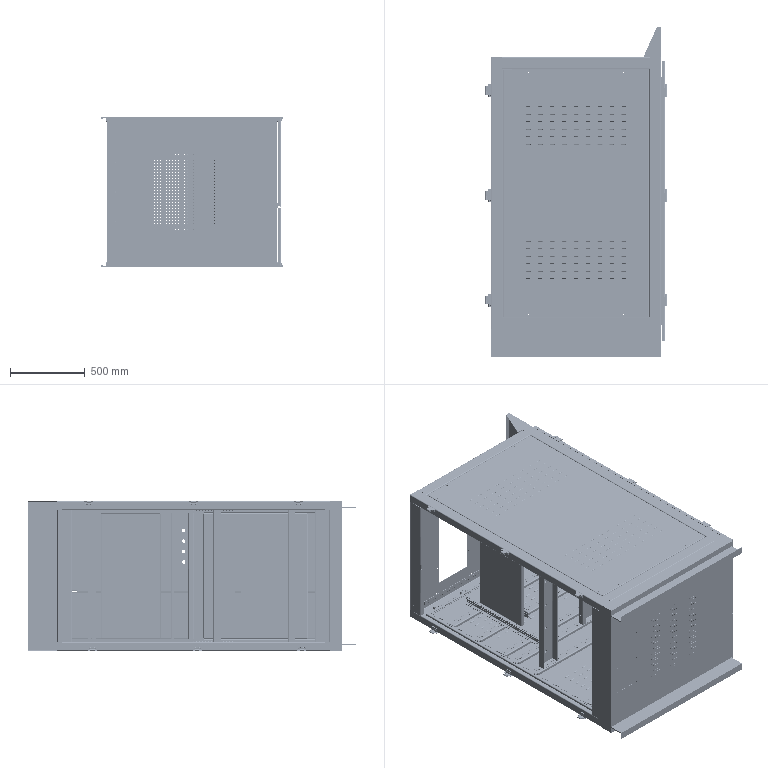Assembly | SolidWorks | mm | 113 component files | 113 solids | 13758 faces | box 1216 x 2200 x 1000 mm | volume 43776213 mm3 | cylinder 8078 | plane 4236 | sphere 864 | torus 432 | spline 100 | cone 48 | commonest cylinder face diameters 9 x4179 5 x1439 12 x336 6 x318 4 x286 16 x216 10 x210 14 x194
Bill of materials:
ACBMountingPlateF5 | 1 |  | Tall rectangular shallow tray/panel with bent perimeter flanges; flanges carry small holes along one long edge and on the short ends.
BaseCover | 1 |  | Rectangular flat panel with shallow return flanges around its edges and six round holes near the two long edges.
BottomSealingPlate | 1 |  | Thin flat rectangular sheet with a rectangular through-cutout, six small holes around the cutout, and a rectangular grid of small perforations.
10#ChannelSteel2 | 2 |  | Long straight U-shaped (channel) profile with no visible holes.
8#ChannelSteel1 | 2 |  | Long C-shaped channel with round holes in its web.
8#ChannelSteel2 | 2 |  | Long inverted-U channel whose top plate extends past the legs at both ends as flat tabs; one leg has a row of six round holes.
8#ChannelSteel3 | 2 |  | Long inverted-U channel similar to the previous part, with top-plate end tabs and two groups of four obround slots in one leg.
8#ChannelSteel5 | 1 |  | Plain long C-shaped channel with no visible holes.
BeamF1 | 12 |  | Long, shallow hat/U-shaped rail with rounded bends; the top web has a continuous row of round holes, and flat end tabs each carry two slots or holes.
BottomBeam | 1 |  | Tall bent sheet-metal profile: a C-section with rounded bends, unequal flanges and a return lip on one flange, with small holes and a small rectangular cutout.
BottomFrameCornerConnection | 2 |  | Flat L-shaped plate with rounded outer corners, a small inner-corner radius and three round through-holes.
Brow | 1 |  | Tall angled sheet-metal cover or wedge shape: two faces meet along a vertical edge, giving a right-trapezoid side profile; one face has small holes and slots.
CapacitorBeamF6 | 2 |  | Long, narrow rectangular tray or trough shape with an open face and closed end walls. It looks like a formed sheet channel.
CapacitorMountingPlateF6-00 | 1 |  | Flat rectangular sheet panel with formed C-shaped return flanges along two opposite edges.
Cover | 1 |  | Flat rectangular plate with one large rectangular cutout set off to one side and holes around the edge.
GL213-1Hinge1 | 6 |  | Block-shaped bracket with two raised, rounded lugs, each with a round through-bore, at either end of a lower connecting bar. It looks like a hinge-knuckle shape.
LeftFrontDoorPanel07-01 | 1 |  | Long, flat rectangular plate with two stacked rectangular windows, a column of round holes, a small slot near the bottom edge, and small hole pairs along the top edge.
MainMountingPlateF4-00 | 1 |  | Nearly square sheet panel with formed return flanges on two opposite edges and one long, narrow through-slot.
MiddleColumnF2-01 | 2 |  | Straight, perforated C-channel (U-channel) with rounded bends and evenly spaced round holes along the web and both flanges.
MiddleColumnF2 | 4 |  | Longer, perforated C-channel with the same profile as the shorter perforated channel. It has evenly spaced round holes along the web and flanges.
MirrorBottomBeam | 1 |  | Long formed sheet channel with an uneven C profile: one flange is short and one is long and ends in a return lip. A few holes run along one face.
MirrorBottomFrameCornerConnection | 2 |  | Flat L-shaped plate with rounded outer corners, a small inside corner radius, and three round through-holes.
MirrorTopBeamConnectionPlate | 2 |  | Flat L-shaped plate with rounded corners and three round through-holes. Its shape is similar to the other L-plate but in a different orientation, possibly mirrored.
MirrorUpperBeam | 1 |  | Long formed sheet post with a stepped profile: a box-like C-section plus an offset side flange. It has a row of small holes along one narrow face, a few larger holes, a small rectangular cutout or tab, and a hole near one end.
ProtectivePlate | 1 |  | Tall, narrow formed sheet-metal panel with several bends. A long flat web is bent into an angled upper section with a short vertical end lip. At the bottom is a horizontal foot leg with a small tab carrying one hole. One long edge flange has a row of small holes.
DoorRearVerticalStiffener06-1 | 2 |  | Long, slender formed rail with an open stepped profile that has rounded bends: a horizontal top flange, a vertical web, a horizontal step and a vertical lower leg. Many evenly spaced small holes run along its length, and there are small notches near the ends.
RightFrontDoorHorizontalStiffener06-02 | 2 |  | Short, straight formed channel section with an open multi-bend profile: two parallel long faces joined by a web, with an offset outer flange and rounded bends. One face has a column of larger round holes and the adjacent offset flange has two smaller holes.
RightFrontDoorPanel06-03 | 1 |  | Long, flat rectangular sheet panel with a narrow, slightly offset flange along one long edge. That flange is shorter than the panel at both ends. Small paired holes sit near the opposite long edge at three locations along the length.
BindingWireRack | 24 |  | U-shaped formed strap: a flat rectangular top web with one central round through-hole, and two parallel legs bent down at rounded corners.
GL213-1Hinge2 | 12 |  | Hinge-leaf-like bracket: a flat base plate with an upright plate that has two round holes and chamfered top corners. Along one edge is a cylindrical barrel (knuckle) with an axial through-bore, connected by a curved transition.
HBSW.001.001ColumnA | 2 |  | Long formed rail with an open profile: a deep C-section with rounded bends, plus a Z-offset step to an extra outward flange. One narrow flange has a dense row of small holes or slots along its length, and the web has a few small hole pairs and end holes.
HBSW.001.002ColumnB | 2 |  | Long formed rail similar in form to unnamed part but with the profile mirrored: an offset Z-step flange joined to a C-like section with rounded bends. One flange has a dense row of perforations, and there are small paired holes at three locations on the web.
HBSW.001.003SideTopBeam | 2 |  | Long formed rail with a multi-bend open profile (several 90-degree rounded bends, including a Z-step). The end tabs extend beyond the main body and carry round holes. One flange has a row of slotted/oblong perforations, and the web has a row of small holes with a few larger ones.
HBSW.001.004SideBottomBeam | 2 |  | Long formed rail with a C-section and a Z-offset extra flange, all with rounded bends. The outer web has six widely spaced elongated slots, the offset flange has a dense row of round holes, and the end tabs carry pairs of small holes.
LiftingRingReinforcementPlate | 4 |  | L-shaped angle bracket with a rounded inside bend. One leg has three equal round holes in a line. The other leg has a large central round hole flanked by two smaller round holes.
SidePlate | 2 |  | Thin, flat rectangular plate with two separate rectangular arrays of short slot-like features (about 9 columns by 6 rows each) near opposite ends, and small holes spaced around the perimeter.
SupportBeamF7 | 2 |  | Long, slender, straight bar or rail that looks like formed sheet. It has a single evenly spaced row of small round holes running along one narrow face. The end view shows a closed or channel-like profile with faceted, bent-looking corners and two large round holes on the end face.
TopBeamConnectionPlate | 2 |  | Flat L-shaped plate of uniform thin thickness with three round through-holes: one near the corner, one at the end of the short leg, and one near the end of the long leg. Outer corners are rounded and the inside corner has a fillet.
UpperBeam | 1 |  | Long, straight, formed sheet profile with a constant cross-section. The section is roughly C-shaped: a long back wall, a top web, a short return flange at the bottom, and on the other side a downward step that ends in an outward flange, with rounded bends. One narrow flange has a long row of small holes with a few larger holes spaced among them. There is a single hole near one end on another face and a small notch partway along one edge.
Mates:
1. coincident | BaseAssembly-1/ChannelSteelAssembly-1/8#ChannelSteel2-2 face at (-409.218, -82.9, -600) dir (0, 0, -1) | SidePanelAssembly-1/HBSW.001.001ColumnA-1 face at (-337.218, 1817.1, -600) dir (0, 0, -1)
2. coincident | BaseAssembly-1/ChannelSteelAssembly-1/8#ChannelSteel2-2 face at (-409.218, -2.9, -600) dir (0, 1, 0) | SidePanelAssembly-1/HBSW.001.004SideBottomBeam-1 face at (-413.718, -2.9, -600) dir (0, -1, 0)
3. coincident | BaseAssembly-1/ChannelSteelAssembly-1/8#ChannelSteel1-2 face at (722.782, -82.9, -600) dir (1, 0, 0) | SidePanelAssembly-1/HBSW.001.002ColumnB-1 face at (722.782, 1817.1, -597) dir (1, 0, 0)
4. coincident | BaseAssembly-1/ChannelSteelAssembly-1/8#ChannelSteel1-1 face at (-417.218, -82.9, 400) dir (-1, 0, 0) | SidePanelAssembly-2/HBSW.001.002ColumnB-1 face at (-417.218, 1817.1, 397) dir (-1, 0, 0)
5. coincident | BaseAssembly-1/ChannelSteelAssembly-1/8#ChannelSteel2-1 face at (714.782, -2.9, 400) dir (0, 1, 0) | SidePanelAssembly-2/HBSW.001.004SideBottomBeam-1 face at (719.282, -2.9, 400) dir (0, -1, 0)
6. coincident | BaseAssembly-1/ChannelSteelAssembly-1/8#ChannelSteel2-1 face at (714.782, -82.9, 400) dir (0, 0, 1) | SidePanelAssembly-2/HBSW.001.004SideBottomBeam-1 face at (-339.718, 77.1, 400) dir (0, 0, 1)
7. concentric | SidePanelAssembly-2/HBSW.001.004SideBottomBeam-1 face at (-372.218, 17.1, 352) dir (0, 0, -1) r 5.5 | BottomBeamAssembly-1/BottomFrameCornerConnection-2 face at (-372.218, 17.1, 332) dir (0, 0, 1) r 5.75
8. concentric | SidePanelAssembly-2/HBSW.001.004SideBottomBeam-1 face at (-397.218, 17.1, 352) dir (0, 0, -1) r 5.5 | BottomBeamAssembly-1/BottomFrameCornerConnection-2 face at (-397.218, 17.1, 332) dir (0, 0, 1) r 5.75
9. coincident | SidePanelAssembly-2/HBSW.001.002ColumnB-1 edge at (-411.218, 27.6, 342) dir (0, 1, 0) | BottomBeamAssembly-1/BottomFrameCornerConnection-2 face at (-414.218, 0.09974, 342) dir (0, 0, 1)
10. concentric | SidePanelAssembly-1/HBSW.001.004SideBottomBeam-1 face at (677.782, 17.1, -552) dir (0, 0, 1) r 5.5 | MirrorBottomBeamAssembly-2/MirrorBottomFrameCornerConnection-1 face at (677.782, 17.1, -549) dir (0, 0, 1) r 5.75
11. concentric | SidePanelAssembly-1/HBSW.001.004SideBottomBeam-1 face at (702.782, 17.1, -552) dir (0, 0, 1) r 5.5 | MirrorBottomBeamAssembly-2/MirrorBottomFrameCornerConnection-1 face at (702.782, 17.1, -549) dir (0, 0, 1) r 5.75
12. coincident | SidePanelAssembly-1/HBSW.001.002ColumnB-1 face at (719.782, 1786.6, -542) dir (0, 0, 1) | MirrorBottomBeamAssembly-2/MirrorBottomFrameCornerConnection-1 face at (719.782, 0.09974, -542) dir (0, 0, -1)
13. concentric | SidePanelAssembly-2/HBSW.001.003SideTopBeam-1 face at (-357.218, 1797.1, 352) dir (0, 0, -1) r 5.5 | TopBeamAssembly-1/TopBeamConnectionPlate-2 face at (-357.218, 1797.1, 349) dir (0, 0, -1) r 5.75
14. concentric | SidePanelAssembly-2/HBSW.001.003SideTopBeam-1 face at (-397.218, 1797.1, 352) dir (0, 0, -1) r 5.5 | TopBeamAssembly-1/TopBeamConnectionPlate-2 face at (-397.218, 1797.1, 349) dir (0, 0, -1) r 5.75
15. coincident | SidePanelAssembly-2/HBSW.001.003SideTopBeam-1 face at (-413.718, 1787.1, 342) dir (0, 0, -1) | TopBeamAssembly-1/TopBeamConnectionPlate-2 face at (-414.218, 1814.1, 342) dir (0, 0, 1)
16. concentric | SidePanelAssembly-1/HBSW.001.003SideTopBeam-1 face at (702.782, 1797.1, -552) dir (0, 0, 1) r 5.5 | MirrorTopBeamAssembly-2/MirrorTopBeamConnectionPlate-1 face at (702.782, 1797.1, -532) dir (0, 0, -1) r 5.75
17. concentric | SidePanelAssembly-1/HBSW.001.003SideTopBeam-1 face at (662.782, 1797.1, -552) dir (0, 0, 1) r 5.5 | MirrorTopBeamAssembly-2/MirrorTopBeamConnectionPlate-1 face at (662.782, 1797.1, -532) dir (0, 0, -1) r 5.75
18. coincident | SidePanelAssembly-1/HBSW.001.003SideTopBeam-1 face at (719.282, 1787.1, -542) dir (0, 0, 1) | MirrorTopBeamAssembly-2/MirrorTopBeamConnectionPlate-1 face at (719.782, 1814.1, -542) dir (0, 0, -1)
19. distance | SidePlate-1 face at (640.782, 1735.6, -597) dir (1, 0, 0) | SidePanelAssembly-1/HBSW.001.002ColumnB-1 face at (642.782, 77.6, -597) dir (-1, 0, 0)
20. distance | SidePanelAssembly-1/HBSW.001.004SideBottomBeam-1 face at (-339.718, 77.1, -597) dir (0, 1, 0) | SidePlate-1 face at (636.782, 78.6, -597) dir (0, -1, 0)
21. coincident | SidePanelAssembly-1/HBSW.001.001ColumnA-1 face at (-337.218, 77.6, -578) dir (0, 0, -1) | SidePlate-1 face at (-335.218, 1735.6, -578) dir (0, 0, 1)
22. distance | SidePlate-2 face at (-335.218, 78.6, 378) dir (-1, 0, 0) | SidePanelAssembly-2/HBSW.001.002ColumnB-1 face at (-337.218, 77.6, 397) dir (1, 0, 0)
23. distance | SidePlate-2 face at (636.782, 1735.6, 397) dir (0, 1, 0) | SidePanelAssembly-2/HBSW.001.003SideTopBeam-1 face at (-339.718, 1737.1, 397) dir (0, -1, 0)
24. coincident | SidePanelAssembly-2/HBSW.001.001ColumnA-1 face at (642.782, 77.6, 378) dir (0, 0, 1) | SidePlate-2 face at (640.782, 78.6, 378) dir (0, 0, -1)
25. distance | Cover-1 face at (640.782, 1790.1, 340) dir (0, 0, 1) | SidePanelAssembly-2/HBSW.001.003SideTopBeam-1 face at (-413.718, 1787.1, 342) dir (0, 0, -1)
26. distance | Cover-1 face at (-335.218, 1790.1, 336) dir (-1, 0, 0) | TopBeamAssembly-1/UpperBeam-1 face at (-337.218, 1817.1, 342) dir (1, 0, 0)
27. coincident | MirrorTopBeamAssembly-2/MirrorUpperBeam-1 face at (642.782, 1790.1, -542) dir (0, 1, 0) | Cover-1 face at (-335.218, 1790.1, -540) dir (0, -1, 0)
28. concentric | SidePanelAssembly-2/GL213-1Hinge2-1 face at (754.782, 1597.1, 394) dir (0, -1, 0) r 3 | LeftFrontDoorAssembly-1/GL213-1Hinge1-1 face at (754.782, 1612.1, 394) dir (0, -1, 0) r 3
29. coincident | SidePanelAssembly-2/GL213-1Hinge2-1 face at (754.782, 1597.1, 400) dir (0, 1, 0) | LeftFrontDoorAssembly-1/GL213-1Hinge1-1 face at (814.782, 1597.1, 400) dir (0, -1, 0)
30. concentric | SidePanelAssembly-1/GL213-1Hinge2-5 face at (754.782, 1592.1, -594) dir (0, 1, 0) r 3 | RightFrontDoorAssembly-1/GL213-1Hinge1-3 face at (754.782, 1577.1, -594) dir (0, 1, 0) r 3
31. coincident | SidePanelAssembly-1/GL213-1Hinge2-5 face at (754.782, 1622.1, -600) dir (0, 1, 0) | RightFrontDoorAssembly-1/GL213-1Hinge1-3 face at (814.782, 1622.1, -600) dir (0, -1, 0)
32. coincident | LeftFrontDoorAssembly-1/LeftFrontDoorPanel07-01-1 face at (747.782, 857.1, 98.5) dir (1, 0, 0) | RightFrontDoorAssembly-1/RightFrontDoorPanel06-03-1 face at (747.782, 857.1, -401) dir (1, 0, 0)
33. concentric | SidePanelAssembly-1/HBSW.001.002ColumnB-1 face at (625.282, 257.1, -585) dir (0, 0, 1) r 4.5 | BeamF1-2 face at (625.282, 257.1, -582) dir (0, 0, 1) r 4.5
34. coincident | SidePanelAssembly-1/HBSW.001.002ColumnB-1 face at (642.782, 1736.6, -575) dir (0, 0, 1) | BeamF1-2 face at (152.782, 247.1, -575) dir (0, 0, -1)
35. concentric | SidePanelAssembly-1/HBSW.001.001ColumnA-1 face at (-319.718, 257.1, -585) dir (0, 0, 1) r 4.5 | BeamF1-2 face at (-319.718, 257.1, -582) dir (0, 0, 1) r 4.5
36. coincident | SidePanelAssembly-2/HBSW.001.001ColumnA-1 face at (642.782, 77.6, 375) dir (0, 0, -1) | BeamF1-14 face at (152.782, 247.1, 375) dir (0, 0, 1)
37. concentric | SidePanelAssembly-2/HBSW.001.001ColumnA-1 face at (625.282, 257.1, 385) dir (0, 0, -1) r 4.5 | BeamF1-14 face at (625.282, 257.1, 382) dir (0, 0, -1) r 4.5
38. concentric | SidePanelAssembly-2/HBSW.001.002ColumnB-1 face at (-319.718, 257.1, 385) dir (0, 0, -1) r 4.5 | BeamF1-14 face at (-319.718, 257.1, 382) dir (0, 0, -1) r 4.5
39. coincident | BeamF1-15 face at (152.782, 747.1, 372) dir (0, 0, -1) | MiddleColumnF2-1 face at (517.782, 497.1, 372) dir (0, 0, 1)
40. concentric | BeamF1-15 face at (532.782, 747.1, 382) dir (0, 0, -1) r 4.5 | MiddleColumnF2-1 face at (532.782, 747.1, 372) dir (0, 0, -1) r 4.5
41. concentric | BeamF1-14 face at (532.782, 247.1, 382) dir (0, 0, -1) r 4.5 | MiddleColumnF2-1 face at (532.782, 247.1, 372) dir (0, 0, -1) r 4.5
42. distance | ACBMountingPlateF5-1 face at (452.782, 942.1, -571) dir (0, 0, -1) | BeamF1-7 face at (152.782, 927.1, -572) dir (0, 0, 1)
43. concentric | BeamF1-16 face at (572.782, 927.1, 382) dir (0, 0, -1) r 4.5 | ACBMountingPlateF5-1 face at (572.782, 927.1, 371.008) dir (0, 0, -1) r 4.5
44. concentric | BeamF1-16 face at (452.782, 927.1, 382) dir (0, 0, -1) r 4.5 | ACBMountingPlateF5-1 face at (452.782, 927.1, 371.008) dir (0, 0, -1) r 4.5
45. distance | CapacitorBeamF6-1 face at (-177.218, 275.1, -571) dir (0, 0, -1) | BeamF1-2 face at (152.782, 247.1, -572) dir (0, 0, 1)
46. concentric | BeamF1-2 face at (-227.218, 247.1, -582) dir (0, 0, 1) r 4.5 | CapacitorBeamF6-1 face at (-227.218, 247.1, -571.008) dir (0, 0, 1) r 4.5
47. concentric | BeamF1-2 face at (-127.218, 247.1, -582) dir (0, 0, 1) r 4.5 | CapacitorBeamF6-1 face at (-127.218, 247.1, -571.008) dir (0, 0, 1) r 4.5
48. coincident | BeamF1-13 face at (152.782, 1527.1, -572) dir (0, 0, 1) | MiddleColumnF2-3 face at (-52.218, 1237.1, -572) dir (0, 0, -1)
49. concentric | BeamF1-13 face at (-67.218, 1527.1, -582) dir (0, 0, 1) r 4.5 | MiddleColumnF2-3 face at (-67.218, 1527.1, -522) dir (0, 0, -1) r 4.5
50. concentric | BeamF1-9 face at (-67.218, 1047.1, -582) dir (0, 0, 1) r 4.5 | MiddleColumnF2-3 face at (-67.218, 1047.1, -522) dir (0, 0, -1) r 4.5
51. distance | CapacitorMountingPlateF6-00-1 face at (-49.718, 1327.1, -521) dir (0, 0, -1) | MiddleColumnF2-3 face at (-52.218, 1237.1, -522) dir (0, 0, 1)
52. concentric | MiddleColumnF2-3 face at (-67.218, 1487.1, -522) dir (0, 0, -1) r 4.5 | CapacitorMountingPlateF6-00-1 face at (-67.218, 1487.1, -521) dir (0, 0, 1) r 4.5
53. concentric | MiddleColumnF2-3 face at (-67.218, 1167.1, -522) dir (0, 0, -1) r 4.5 | CapacitorMountingPlateF6-00-1 face at (-67.218, 1167.1, -521) dir (0, 0, 1) r 4.5
54. coincident | BeamF1-13 face at (152.782, 1527.1, -572) dir (0, 0, 1) | MiddleColumnF2-01-1 face at (97.782, 1417.1, -572) dir (0, 0, -1)
55. concentric | BeamF1-12 face at (112.782, 1287.1, -582) dir (0, 0, 1) r 4.5 | MiddleColumnF2-01-1 face at (112.782, 1287.1, -572) dir (0, 0, 1) r 4.5
56. concentric | BeamF1-13 face at (112.782, 1527.1, -582) dir (0, 0, 1) r 4.5 | MiddleColumnF2-01-1 face at (112.782, 1527.1, -572) dir (0, 0, 1) r 4.5
57. distance | SupportBeamF7-1 face at (142.782, 1059.1, -571) dir (0, 0, -1) | BeamF1-9 face at (152.782, 1047.1, -572) dir (0, 0, 1)
58. concentric | BeamF1-9 face at (152.782, 1047.1, -582) dir (0, 0, 1) r 4.5 | SupportBeamF7-1 face at (152.782, 1047.1, 371.008) dir (0, 0, -1) r 4.5
59. concentric | BeamF1-9 face at (132.782, 1047.1, -582) dir (0, 0, 1) r 4.5 | SupportBeamF7-1 face at (132.782, 1047.1, 371.008) dir (0, 0, -1) r 4.5
60. coincident | MiddleColumnF2-01-2 face at (97.782, 1417.1, 347) dir (-1, 0, 0) | SupportBeamF7-2 face at (97.782, 1587.1, -100) dir (1, 0, 0)
61. concentric | MiddleColumnF2-01-1 face at (107.782, 1587.1, -557) dir (-1, 0, 0) r 4.5 | SupportBeamF7-2 face at (87.782, 1587.1, -557) dir (1, 0, 0) r 4.5
62. concentric | MiddleColumnF2-01-2 face at (107.782, 1587.1, 357) dir (-1, 0, 0) r 4.5 | SupportBeamF7-2 face at (87.782, 1587.1, 357) dir (1, 0, 0) r 4.5
63. coincident | SidePanelAssembly-1/HBSW.001.003SideTopBeam-1 face at (-339.718, 1737.1, -600) dir (0, 0, -1) | Brow-1 face at (722.782, 1917.1, -600) dir (0, 0, -1)
64. coincident | SidePanelAssembly-1/HBSW.001.002ColumnB-1 face at (722.782, 1817.1, -597) dir (1, 0, 0) | Brow-1 face at (722.782, 1917.1, -100) dir (1, 0, 0)
65. coincident | SidePanelAssembly-1/HBSW.001.003SideTopBeam-1 face at (719.282, 1817.1, -600) dir (0, 1, 0) | Brow-1 face at (722.782, 1817.1, -100) dir (0, -1, 0)
66. distance | MainMountingPlateF4-00-3 face at (515.282, 492.1, -521) dir (0, 0, -1) | MiddleColumnF2-2 face at (517.782, 497.1, -522) dir (0, 0, 1)
67. concentric | MiddleColumnF2-2 face at (532.782, 787.1, -522) dir (0, 0, -1) r 4.5 | MainMountingPlateF4-00-3 face at (532.782, 787.1, -521) dir (0, 0, 1) r 4.5
68. concentric | MiddleColumnF2-2 face at (532.782, 487.1, -522) dir (0, 0, -1) r 4.5 | MainMountingPlateF4-00-3 face at (532.782, 487.1, -521) dir (0, 0, 1) r 4.5
69. concentric | ACBMountingPlateF5-1 face at (302.346, 922.1, -100) dir (1, 0, 0) r 4.5 | ProtectivePlate-1 face at (612.782, 922.1, -100) dir (-1, 0, 0) r 4.5
70. concentric | ACBMountingPlateF5-1 face at (302.346, 922.1, -500) dir (1, 0, 0) r 4.5 | ProtectivePlate-1 face at (612.782, 922.1, -500) dir (-1, 0, 0) r 4.5
71. coincident | ACBMountingPlateF5-1 face at (602.782, 942.1, -100) dir (1, 0, 0) | ProtectivePlate-1 face at (602.782, 937.1, 340) dir (-1, 0, 0)
72. coincident | ChannelSteelAssembly-1/8#ChannelSteel3-2 face at (644.857, -90.892, 127.5) dir (0, -1, 0) | BottomSealingPlate-1 face at (-467.143, -90.892, 352) dir (0, 1, 0)
73. coincident | ChannelSteelAssembly-1/10#ChannelSteel2-1 face at (652.857, -190.892, -552) dir (0, 0, 1) | BottomSealingPlate-1 face at (-467.143, -92.892, -552) dir (0, 0, -1)
74. distance | BottomSealingPlate-1 edge at (-467.143, -92.892, 352) dir (0, 0, -1) | ChannelSteelAssembly-1/8#ChannelSteel1-1 face at (-487.143, -90.892, 400) dir (-1, 0, 0)
75. concentric | BottomSealingPlate-1 face at (-428.143, -82.892, 100) dir (0, -1, 0) r 5.5 | BaseCover-1 face at (-428.143, -88.892, 100) dir (0, 1, 0) r 3.5
76. concentric | BottomSealingPlate-1 face at (-428.143, -82.892, -300) dir (0, -1, 0) r 5.5 | BaseCover-1 face at (-428.143, -88.892, -300) dir (0, 1, 0) r 3.5
77. coincident | BottomSealingPlate-1 face at (-467.143, -90.892, 352) dir (0, 1, 0) | BaseCover-1 face at (-434.143, -90.892, -315) dir (0, -1, 0)
78. coincident | 8#ChannelSteel1-1 face at (-30.895, 33.973, 400) dir (1, 0, 0) | 8#ChannelSteel2-1 face at (-30.895, 37.973, 360) dir (-1, 0, 0)
79. coincident | 8#ChannelSteel1-1 face at (-38.895, 37.973, 400) dir (0, 1, 0) | 8#ChannelSteel2-1 face at (1093.105, 37.973, 400) dir (0, 1, 0)
80. coincident | 8#ChannelSteel1-1 face at (1.105, 37.973, 400) dir (0, 0, 1) | 8#ChannelSteel2-1 face at (1093.105, -42.027, 400) dir (0, 0, 1)
81. coincident | 8#ChannelSteel2-1 face at (1093.105, 37.973, 400) dir (0, 1, 0) | 8#ChannelSteel1-2 face at (1101.105, 37.973, -600) dir (0, 1, 0)
82. coincident | 8#ChannelSteel2-1 face at (1093.105, 37.973, 360) dir (1, 0, 0) | 8#ChannelSteel1-2 face at (1093.105, 33.973, -600) dir (-1, 0, 0)
83. coincident | 8#ChannelSteel2-1 face at (1093.105, -42.027, 400) dir (0, 0, 1) | 8#ChannelSteel1-2 face at (1061.105, 37.973, 400) dir (0, 0, 1)
84. coincident | 8#ChannelSteel1-1 face at (-30.895, 33.973, 400) dir (1, 0, 0) | 8#ChannelSteel2-2 face at (-30.895, 37.973, -560) dir (-1, 0, 0)
85. coincident | 8#ChannelSteel1-1 face at (1.105, 37.973, -600) dir (0, 0, -1) | 8#ChannelSteel2-2 face at (-30.895, -42.027, -600) dir (0, 0, -1)
86. coincident | 8#ChannelSteel1-1 face at (-38.895, 37.973, 400) dir (0, 1, 0) | 8#ChannelSteel2-2 face at (-30.895, 37.973, -600) dir (0, 1, 0)
87. coincident | 10#ChannelSteel2-1 face at (1101.105, -42.027, -552) dir (0, 1, 0) | 8#ChannelSteel2-2 face at (-30.895, -42.027, -560) dir (0, -1, 0)
88. coincident | 10#ChannelSteel2-1 face at (1101.105, -42.027, -600) dir (1, 0, 0) | 8#ChannelSteel1-2 face at (1101.105, -42.027, -600) dir (1, 0, 0)
89. coincident | 10#ChannelSteel2-1 face at (1101.105, -42.027, -600) dir (0, 0, -1) | 8#ChannelSteel2-2 face at (-30.895, -42.027, -600) dir (0, 0, -1)
90. coincident | 8#ChannelSteel2-1 face at (1093.105, -42.027, 360) dir (0, -1, 0) | 10#ChannelSteel2-2 face at (-38.895, -42.027, 352) dir (0, 1, 0)
91. coincident | 8#ChannelSteel1-1 face at (-38.895, -42.027, 400) dir (-1, 0, 0) | 10#ChannelSteel2-2 face at (-38.895, -42.027, 400) dir (-1, 0, 0)
92. coincident | 8#ChannelSteel2-1 face at (1093.105, -42.027, 400) dir (0, 0, 1) | 10#ChannelSteel2-2 face at (-38.895, -42.027, 400) dir (0, 0, 1)
93. coincident | 8#ChannelSteel1-2 face at (1093.105, 33.973, -600) dir (-1, 0, 0) | 8#ChannelSteel3-1 face at (1093.105, 37.973, -367.5) dir (1, 0, 0)
94. coincident | 8#ChannelSteel1-2 face at (1101.105, 37.973, -600) dir (0, 1, 0) | 8#ChannelSteel3-1 face at (1093.105, 37.973, -327.5) dir (0, 1, 0)
95. coincident | 8#ChannelSteel5-1 face at (251.105, 37.973, -327.5) dir (0, 1, 0) | 8#ChannelSteel3-1 face at (1093.105, 37.973, -327.5) dir (0, 1, 0)
96. coincident | 8#ChannelSteel5-1 face at (251.105, -42.027, -327.5) dir (0, 0, -1) | 8#ChannelSteel3-1 face at (1093.105, -42.027, -327.5) dir (0, 0, 1)
97. coincident | 8#ChannelSteel5-1 face at (251.105, -42.027, 127.5) dir (0, 0, 1) | 8#ChannelSteel3-2 face at (1093.105, 37.973, 127.5) dir (0, 0, -1)
98. coincident | 8#ChannelSteel5-1 face at (251.105, 37.973, -327.5) dir (0, 1, 0) | 8#ChannelSteel3-2 face at (1093.105, 37.973, 167.5) dir (0, 1, 0)
99. coincident | 8#ChannelSteel1-1 face at (-30.895, 33.973, 400) dir (1, 0, 0) | 8#ChannelSteel3-2 face at (-30.895, -42.027, 167.5) dir (-1, 0, 0)
100. distance | 8#ChannelSteel5-1 face at (211.105, 37.973, -327.5) dir (-1, 0, 0) | 8#ChannelSteel1-1 face at (-30.895, 33.973, 400) dir (1, 0, 0)
101. distance | 8#ChannelSteel3-1 face at (1093.105, 33.973, -335.5) dir (0, 0, -1) | 8#ChannelSteel2-2 face at (-30.895, 33.973, -592) dir (0, 0, 1)
102. coincident | BottomBeam-1 face at (50.625, 24.119, 342) dir (-1, 0, 0) | BottomFrameCornerConnection-1 face at (50.625, 21.119, 342) dir (1, 0, 0)
103. coincident | BottomBeam-1 face at (53.625, 21.119, 342) dir (0, -1, 0) | BottomFrameCornerConnection-1 face at (-43.375, 21.119, 342) dir (0, 1, 0)
104. coincident | BottomBeam-1 face at (-43.375, 18.119, 342) dir (0, 0, 1) | BottomFrameCornerConnection-1 face at (50.625, 21.119, 342) dir (0, 0, 1)
105. concentric | GL213-1Hinge1-1 face at (176.406, 371.994, 16.497) dir (0, 0, -1) r 3 | LeftFrontDoorPanel07-01-1 face at (176.406, 371.994, 1.498) dir (0, 0, 1) r 3
106. concentric | GL213-1Hinge1-1 face at (176.406, 361.994, 16.497) dir (0, 0, -1) r 3 | LeftFrontDoorPanel07-01-1 face at (176.406, 361.994, 1.498) dir (0, 0, 1) r 3
107. coincident | LeftFrontDoorPanel07-01-1 face at (459.506, -375.506, 11.498) dir (0, 0, 1) | GL213-1Hinge1-1 face at (182.606, 319.494, 11.498) dir (0, 0, -1)
108. coincident | MirrorBottomBeam-1 face at (50.625, 24.119, -342) dir (-1, 0, 0) | MirrorBottomFrameCornerConnection-1 face at (50.625, 21.119, -342) dir (1, 0, 0)
109. coincident | MirrorBottomBeam-1 face at (53.625, 21.119, -342) dir (0, -1, 0) | MirrorBottomFrameCornerConnection-1 face at (-43.375, 21.119, -342) dir (0, 1, 0)
110. coincident | MirrorBottomBeam-1 face at (-43.375, 18.119, -342) dir (0, 0, -1) | MirrorBottomFrameCornerConnection-1 face at (50.625, 21.119, -342) dir (0, 0, -1)
111. coincident | MirrorUpperBeam-1 face at (41.857, 57.751, -342) dir (0, -1, 0) | MirrorTopBeamConnectionPlate-1 face at (-55.143, 57.751, 539) dir (0, 1, 0)
112. coincident | MirrorUpperBeam-1 face at (38.857, 60.751, -342) dir (-1, 0, 0) | MirrorTopBeamConnectionPlate-1 face at (38.857, 57.751, 539) dir (1, 0, 0)
113. coincident | MirrorUpperBeam-1 face at (-52.143, 54.751, 542) dir (0, 0, 1) | MirrorTopBeamConnectionPlate-1 face at (38.857, 57.751, 542) dir (0, 0, 1)
114. coincident | RightFrontDoorPanel06-03-1 face at (-537.577, -123.648, 10.497) dir (0, 0, -1) | DoorRearVerticalStiffener06-1-1 face at (-414.577, -123.648, 10.497) dir (0, 0, 1)
115. coincident | RightFrontDoorPanel06-03-1 face at (-537.577, 809.352, 12.497) dir (0, -1, 0) | DoorRearVerticalStiffener06-1-1 face at (-424.577, 809.352, 10.497) dir (0, 1, 0)
116. distance | DoorRearVerticalStiffener06-1-1 face at (-404.577, -123.648, -7.503) dir (1, 0, 0) | RightFrontDoorPanel06-03-1 face at (-344.577, -123.648, 12.497) dir (-1, 0, 0)
117. coincident | RightFrontDoorPanel06-03-1 face at (-537.577, -123.648, 10.497) dir (0, 0, -1) | RightFrontDoorHorizontalStiffener06-02-1 face at (-539.577, 749.352, 10.497) dir (0, 0, 1)
118. coincident | RightFrontDoorHorizontalStiffener06-02-1 face at (-539.577, 759.352, -7.503) dir (0, 1, 0) | DoorRearVerticalStiffener06-1-1 face at (-439.577, 759.352, 10.497) dir (0, -1, 0)
119. coincident | RightFrontDoorHorizontalStiffener06-02-1 face at (-424.577, 759.352, -6.503) dir (1, 0, 0) | DoorRearVerticalStiffener06-1-1 face at (-424.577, -123.648, -7.503) dir (-1, 0, 0)
120. coincident | RightFrontDoorPanel06-03-1 face at (-537.577, -123.648, 10.497) dir (0, 0, -1) | RightFrontDoorHorizontalStiffener06-02-2 face at (-539.577, -996.648, 10.497) dir (0, 0, 1)
121. coincident | DoorRearVerticalStiffener06-1-1 face at (-414.577, -1006.648, 9.497) dir (0, 1, 0) | RightFrontDoorHorizontalStiffener06-02-2 face at (-539.577, -1006.648, -7.503) dir (0, -1, 0)
122. coincident | DoorRearVerticalStiffener06-1-1 face at (-424.577, -123.648, -7.503) dir (-1, 0, 0) | RightFrontDoorHorizontalStiffener06-02-2 face at (-424.577, -986.648, -6.503) dir (1, 0, 0)
123. coincident | RightFrontDoorPanel06-03-1 face at (-537.577, -123.648, 10.497) dir (0, 0, -1) | DoorRearVerticalStiffener06-1-2 face at (-664.577, -123.648, 10.497) dir (0, 0, 1)
124. coincident | RightFrontDoorPanel06-03-1 face at (-537.577, -1056.648, 12.497) dir (0, 1, 0) | DoorRearVerticalStiffener06-1-2 face at (-654.577, -1056.648, 10.497) dir (0, -1, 0)
125. coincident | RightFrontDoorHorizontalStiffener06-02-2 face at (-654.577, -1006.648, 10.497) dir (-1, 0, 0) | DoorRearVerticalStiffener06-1-2 face at (-654.577, -123.648, -7.503) dir (1, 0, 0)
126. concentric | RightFrontDoorPanel06-03-1 face at (-718.177, 548.852, 2.497) dir (0, 0, 1) r 3 | GL213-1Hinge1-1 face at (-718.177, 548.852, 17.497) dir (0, 0, -1) r 3
127. concentric | RightFrontDoorPanel06-03-1 face at (-718.177, 538.852, 2.497) dir (0, 0, 1) r 3 | GL213-1Hinge1-1 face at (-718.177, 538.852, 17.497) dir (0, 0, -1) r 3
128. coincident | RightFrontDoorPanel06-03-1 face at (-537.577, -123.648, 12.497) dir (0, 0, 1) | GL213-1Hinge1-1 face at (-711.977, 496.352, 12.497) dir (0, 0, -1)
129. coincident | HBSW.001.002ColumnB-1 face at (896.246, 860.172, -29) dir (0, 0, -1) | HBSW.001.003SideTopBeam-1 face at (-843.754, -122.328, -29) dir (0, 0, -1)
130. coincident | HBSW.001.002ColumnB-1 face at (-923.754, 940.172, 29) dir (-1, 0, 0) | HBSW.001.003SideTopBeam-1 face at (-923.754, 936.672, -29) dir (-1, 0, 0)
131. distance | HBSW.001.002ColumnB-1 face at (-923.754, 937.172, -26) dir (0, -1, 0) | HBSW.001.003SideTopBeam-1 face at (-923.754, 936.672, 29) dir (0, 1, 0)
132. coincident | HBSW.001.001ColumnA-1 face at (-923.754, -119.828, -29) dir (0, 0, -1) | HBSW.001.003SideTopBeam-1 face at (-843.754, -122.328, -29) dir (0, 0, -1)
133. coincident | HBSW.001.001ColumnA-1 face at (-923.754, -199.828, -26) dir (-1, 0, 0) | HBSW.001.003SideTopBeam-1 face at (-923.754, 936.672, -29) dir (-1, 0, 0)
134. distance | HBSW.001.001ColumnA-1 face at (896.246, -196.828, -26) dir (0, 1, 0) | HBSW.001.003SideTopBeam-1 face at (-923.754, -196.328, 29) dir (0, -1, 0)
135. coincident | HBSW.001.002ColumnB-1 face at (896.246, 860.172, -29) dir (0, 0, -1) | HBSW.001.004SideBottomBeam-1 face at (816.246, 862.672, -29) dir (0, 0, -1)
136. coincident | HBSW.001.002ColumnB-1 face at (896.246, 940.172, -29) dir (1, 0, 0) | HBSW.001.004SideBottomBeam-1 face at (896.246, -196.328, -29) dir (1, 0, 0)
137. distance | HBSW.001.004SideBottomBeam-1 face at (896.246, 936.672, 29) dir (0, 1, 0) | HBSW.001.002ColumnB-1 face at (-923.754, 937.172, -26) dir (0, -1, 0)
138. concentric | HBSW.001.003SideTopBeam-1 face at (-913.754, 895.172, -4) dir (-1, 0, 0) r 7 | LiftingRingReinforcementPlate-1 face at (-910.754, 895.172, -4) dir (-1, 0, 0) r 6.5
139. coincident | HBSW.001.003SideTopBeam-1 face at (-920.754, 936.672, -29) dir (1, 0, 0) | LiftingRingReinforcementPlate-1 face at (-920.754, 860.172, 14) dir (-1, 0, 0)
140. parallel | HBSW.001.003SideTopBeam-1 face at (-893.754, 936.672, 29) dir (0, 0, 1) | LiftingRingReinforcementPlate-1 face at (-917.754, 930.172, 14) dir (0, 0, 1)
141. coincident | HBSW.001.003SideTopBeam-1 face at (-843.754, -122.328, -26) dir (0, 0, 1) | BindingWireRack-1 face at (-877.754, -24.828, -26) dir (0, 0, -1)
142. distance | BindingWireRack-1 face at (-877.754, -24.828, -11) dir (0, -1, 0) | HBSW.001.001ColumnA-1 face at (896.246, -196.828, -26) dir (0, 1, 0)
143. distance | BindingWireRack-1 face at (-862.754, -22.828, -15) dir (1, 0, 0) | HBSW.001.003SideTopBeam-1 face at (-846.754, 862.672, -26) dir (-1, 0, 0)
144. coincident | HBSW.001.001ColumnA-1 face at (-923.754, -119.828, -26) dir (0, 0, 1) | BindingWireRack-9 face at (-715.754, -153.828, -26) dir (0, 0, -1)
145. distance | BindingWireRack-9 face at (-679.754, -138.828, -15) dir (0, 1, 0) | HBSW.001.001ColumnA-1 face at (-843.254, -122.828, -26) dir (0, -1, 0)
146. distance | BindingWireRack-9 face at (-717.754, -153.828, -26) dir (-1, 0, 0) | LiftingRingReinforcementPlate-2 face at (-917.754, -189.828, 14) dir (1, 0, 0)
147. concentric | HBSW.001.001ColumnA-1 face at (-701.254, -189.828, -7.5) dir (0, -1, 0) r 3.5 | GL213-1Hinge2-1 face at (-701.254, -174.828, -7.5) dir (0, -1, 0) r 3.15
148. concentric | HBSW.001.001ColumnA-1 face at (-676.254, -189.828, -7.5) dir (0, -1, 0) r 3.5 | GL213-1Hinge2-1 face at (-676.254, -174.828, -7.5) dir (0, -1, 0) r 3.15
149. coincident | HBSW.001.001ColumnA-1 face at (896.246, -199.828, -26) dir (0, -1, 0) | GL213-1Hinge2-1 face at (-658.754, -199.828, -29) dir (0, 1, 0)
150. concentric | HBSW.001.002ColumnB-1 face at (-726.254, 930.172, -7.5) dir (0, 1, 0) r 3.5 | GL213-1Hinge2-5 face at (-726.254, 915.172, -7.5) dir (0, 1, 0) r 3.15
151. concentric | HBSW.001.002ColumnB-1 face at (-701.254, 930.172, -7.5) dir (0, 1, 0) r 3.5 | GL213-1Hinge2-5 face at (-701.254, 915.172, -7.5) dir (0, 1, 0) r 3.15
152. coincident | HBSW.001.002ColumnB-1 face at (-923.754, 940.172, -26) dir (0, 1, 0) | GL213-1Hinge2-5 face at (-743.754, 940.172, -29) dir (0, -1, 0)
153. coincident | UpperBeam-1 face at (41.857, 57.751, 342) dir (0, -1, 0) | TopBeamConnectionPlate-1 face at (-55.143, 57.751, -539) dir (0, 1, 0)
154. coincident | UpperBeam-1 face at (38.857, 60.751, 342) dir (-1, 0, 0) | TopBeamConnectionPlate-1 face at (38.857, 57.751, -539) dir (1, 0, 0)
155. coincident | UpperBeam-1 face at (-52.143, 54.751, -542) dir (0, 0, -1) | TopBeamConnectionPlate-1 face at (38.857, 57.751, -542) dir (0, 0, -1)